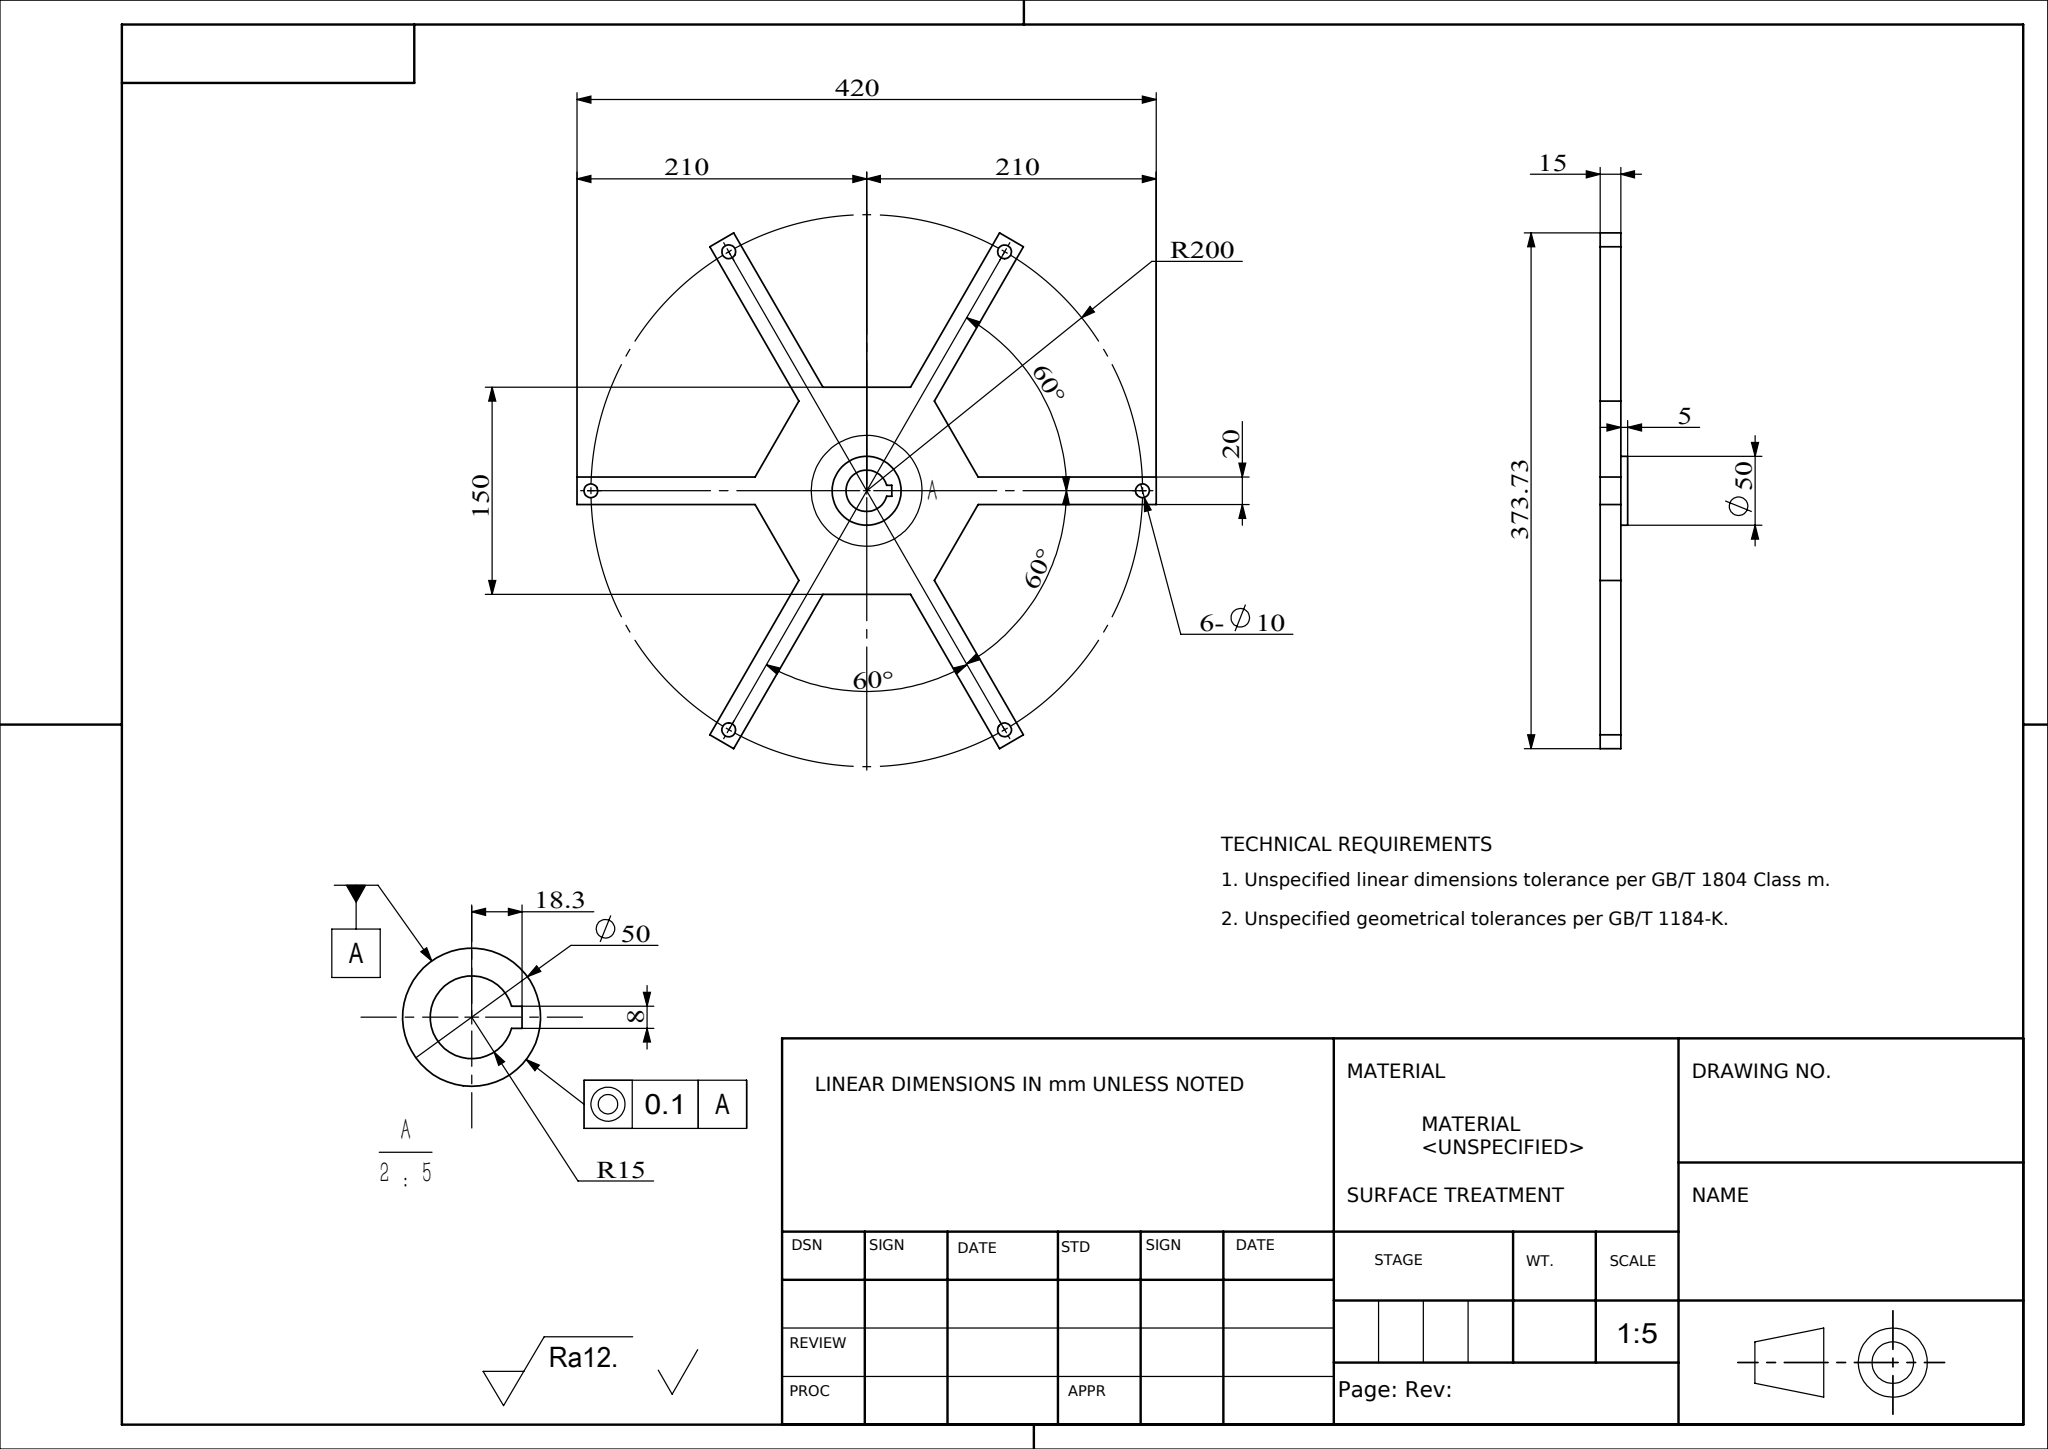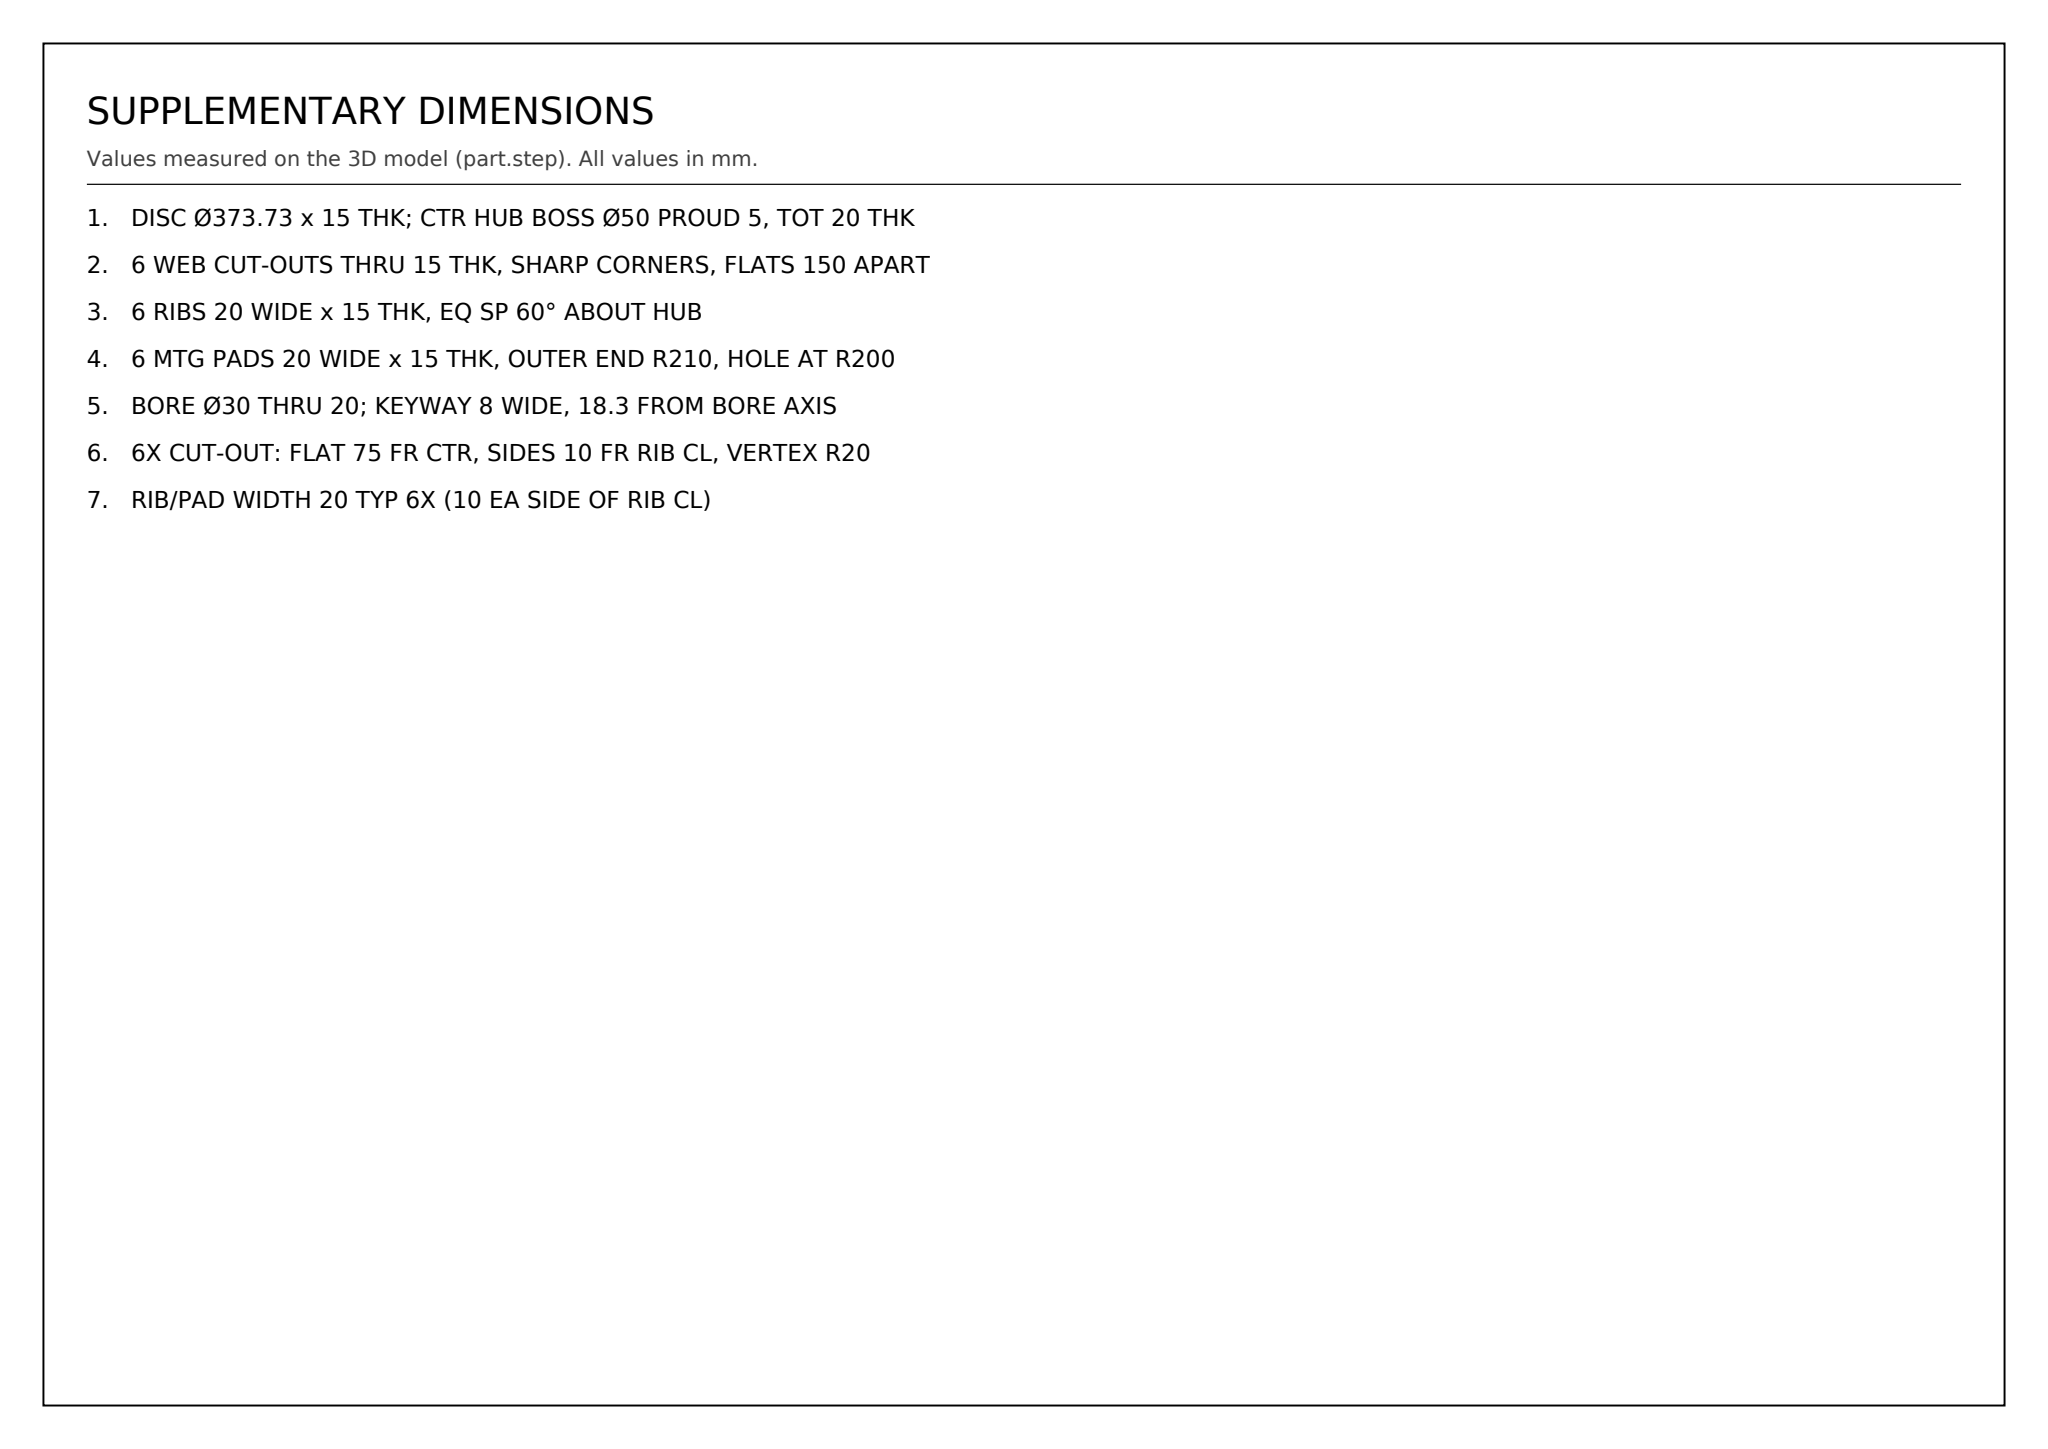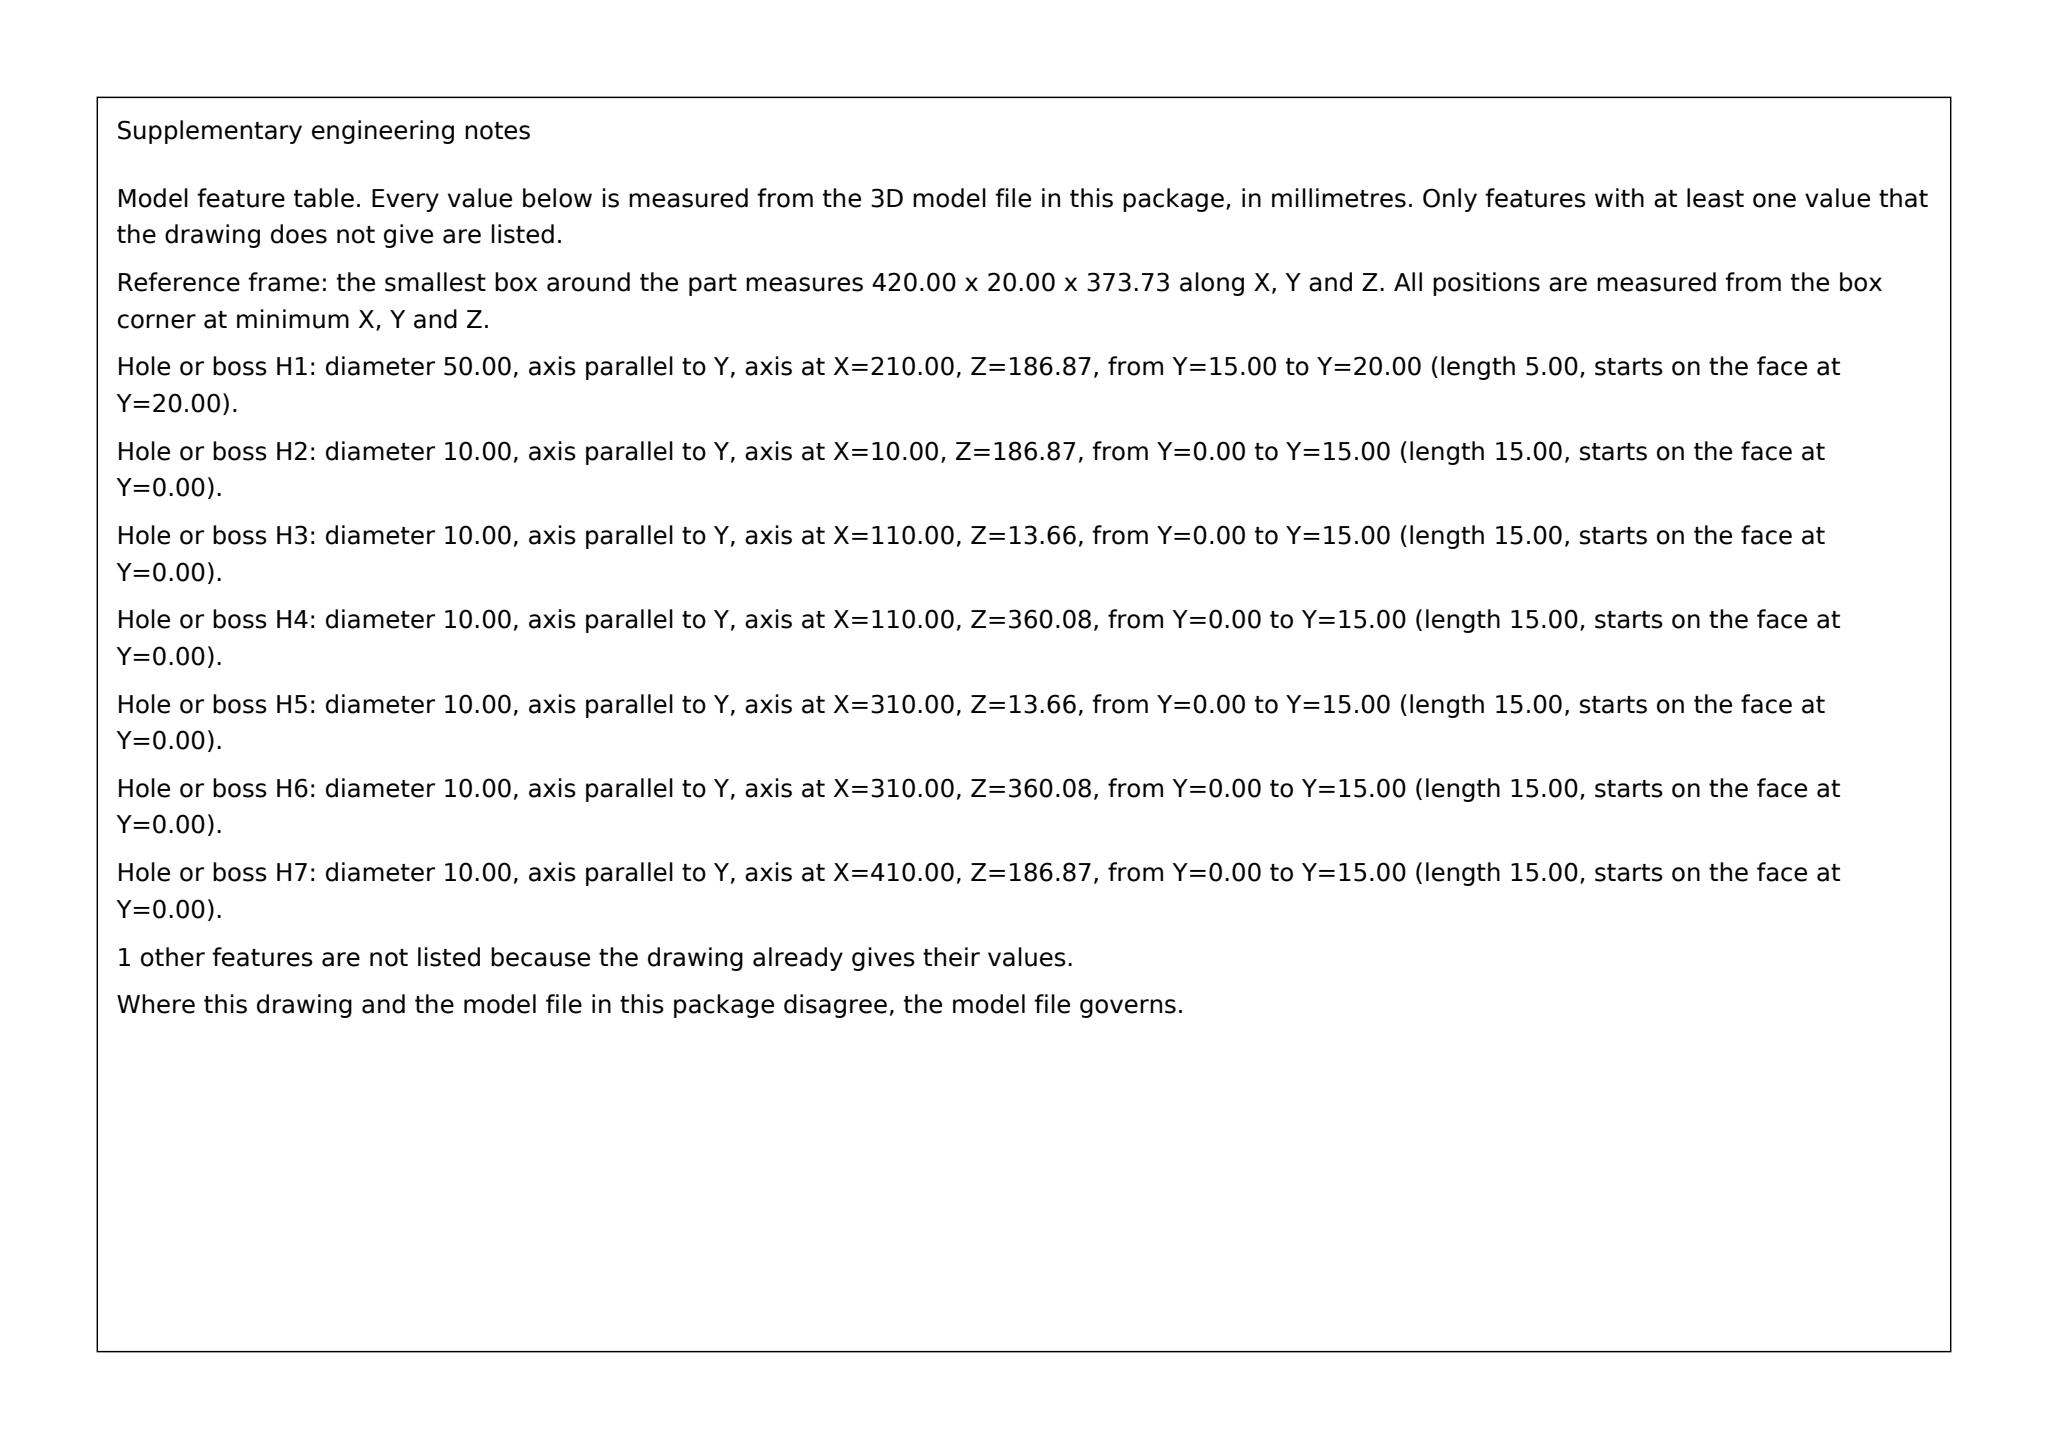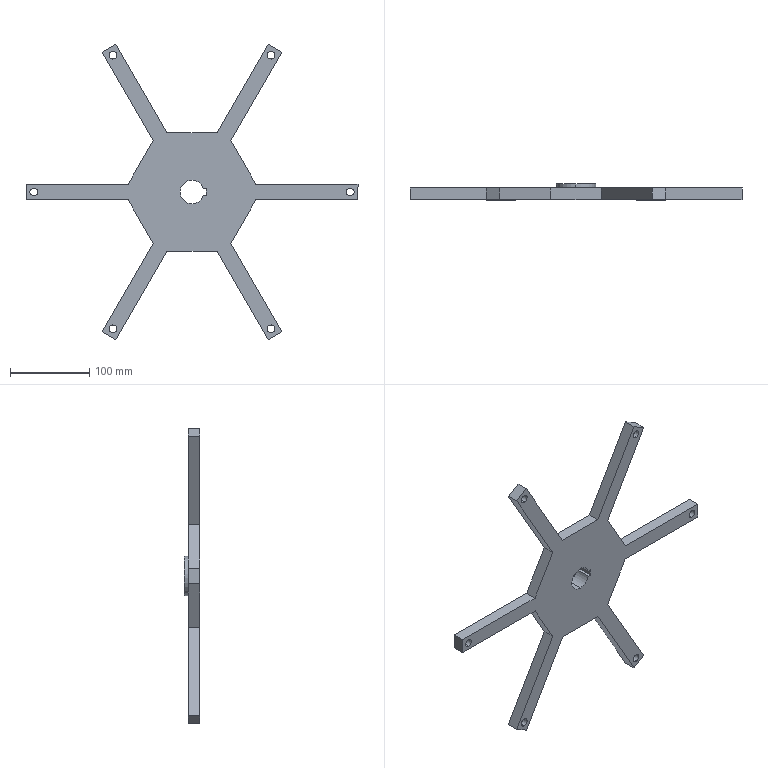Part | SolidWorks | mm | 1 solid | 47 faces | box 420 x 20 x 373.73 mm | volume 507650 mm3 | plane 30 | cylinder 17 | commonest cylinder face diameters 10 x12 30 x3 50 x2
Drawing notes:
DISC Ø373.73 x 15 THK; CTR HUB BOSS Ø50 PROUD 5, TOT 20 THK | from the solid: bbox z=373.731 = disc OD; y planes 0/15/20, bbox y=20; cyl Ø50 axis y len 5 at (210,186.87)
6 WEB CUT-OUTS THRU 15 THK, SHARP CORNERS, FLATS 150 APART | from the solid: fillet_radii [] (no radii); z planes 111.87 & 261.87 = 150 apart, sym about z=186.87; plate 15 thk (y 0-15)
6 RIBS 20 WIDE x 15 THK, EQ SP 60° ABOUT HUB | from the solid: z planes 176.87 & 196.87 straddle rib CL z=186.87 (20 wide); y planes 0/15 = 15 thk; 6-fold Ø10 hole pattern at 60°
6 MTG PADS 20 WIDE x 15 THK, OUTER END R210, HOLE AT R200 | from the solid: pad side planes z=176.87/196.87 (20 wide); x plane 420 = 210 from CL x=210; Ø10 holes at R200 from (210,186.87)
BORE Ø30 THRU 20; KEYWAY 8 WIDE, 18.3 FROM BORE AXIS | from the solid: cyl Ø30 (R15) axis y len 20; keyway faces z=182.87/190.87 (8 wide); end plane x=228.3 = 18.3 from axis x=210
6X CUT-OUT: FLAT 75 FR CTR, SIDES 10 FR RIB CL, VERTEX R20 | from the solid: z planes 111.87 & 261.87 = +/-75 from hub CL z=186.87 (150 apart); z planes 176.87/196.87 = +/-10 from rib CL; ribs 60 deg apart -> inner vertex at R20
RIB/PAD WIDTH 20 TYP 6X (10 EA SIDE OF RIB CL) | from the solid: axis_planes z 176.87 & 196.87 (count 2 each) = 20 wide about hub CL z=186.87; 6 ribs to 6X dia10 holes at R200
build123d program:
from build123d import *

# Parameters (mm, degrees)
BOSS_EXTRUDE1_DEPTH = 15
SKETCH2_R           = 15
CUT_EXTRUDE1_DEPTH  = 20
BOSS_EXTRUDE2_DEPTH = 15
SKETCH4_R           = 5
CUT_EXTRUDE2_DEPTH  = 20
CIRPATTERN1_COUNT   = 6
BOSS_EXTRUDE3_START = 5
SKETCH5_R           = 25
SKETCH5_R_2         = 15
BOSS_EXTRUDE3_DEPTH = 5
SKETCH6_W           = 18.3
SKETCH6_H           = 8
CUT_EXTRUDE3_DEPTH  = 282.813


with BuildPart() as part:
    # Sketch1 → Boss-Extrude1 (new body)
    with BuildSketch(Plane(origin=(0, 0, 0), x_dir=(1, 0, 0), z_dir=(0, 1, 0))):
        Polygon((86.603, 0), (43.301, 75), (-43.301, 75), (-86.603, 0), (-43.301, -75), (43.301, -75), align=None)
    extrude(amount=BOSS_EXTRUDE1_DEPTH)

    # Sketch2 → Cut-Extrude1 (cut)
    with BuildSketch(Plane(origin=(0, 15, 0), x_dir=(1, 0, 0), z_dir=(0, 1, 0))):
        with Locations(Location((0, 0, 0), (0, 0, 270))):
            Circle(SKETCH2_R)
    extrude(amount=-CUT_EXTRUDE1_DEPTH, mode=Mode.SUBTRACT)

    # Sketch3 → Boss-Extrude2 (add)
    with BuildSketch(Plane(origin=(0, 15, 0), x_dir=(1, 0, 0), z_dir=(0, 1, 0))):
        Polygon((24.096, 61.736), (96.34, 186.865), (113.66, 176.865), (41.417, 51.736), align=None)
    boss_extrude2 = extrude(amount=-BOSS_EXTRUDE2_DEPTH)

    # Sketch4 → Cut-Extrude2 (cut)
    with BuildSketch(Plane(origin=(0, 15, 0), x_dir=(1, 0, 0), z_dir=(0, 1, 0))):
        with Locations(Location((100, 173.205, 0), (0, 0, 270))):
            Circle(SKETCH4_R)
    cut_extrude2 = extrude(amount=-CUT_EXTRUDE2_DEPTH, mode=Mode.SUBTRACT)

    # CirPattern1: Boss-Extrude2, Cut-Extrude2 ×6 about axis
    cirpattern1_axis = Axis((0, 0, 0), (0, 1, 0))
    add([boss_extrude2.rotate(cirpattern1_axis, i * 360 / CIRPATTERN1_COUNT) for i in range(1, CIRPATTERN1_COUNT)])
    add([cut_extrude2.rotate(cirpattern1_axis, i * 360 / CIRPATTERN1_COUNT) for i in range(1, CIRPATTERN1_COUNT)], mode=Mode.SUBTRACT)

    # Sketch5 → Boss-Extrude3 (add)
    with BuildSketch(Plane(origin=(0, 15, 0), x_dir=(1, 0, 0), z_dir=(0, 1, 0)).offset(BOSS_EXTRUDE3_START)):
        with Locations(Location((0, 0, 0), (0, 0, 270))):
            Circle(SKETCH5_R)
        with Locations(Location((0, 0, 0), (0, 0, 270))):
            Circle(SKETCH5_R_2, mode=Mode.SUBTRACT)
    extrude(amount=-BOSS_EXTRUDE3_DEPTH)

    # Sketch6 → Cut-Extrude3 (cut, through all)
    with BuildSketch(Plane(origin=(0, 20, 0), x_dir=(1, 0, 0), z_dir=(0, 1, 0))):
        with Locations((9.15, 0)):
            Rectangle(SKETCH6_W, SKETCH6_H)
    extrude(amount=-CUT_EXTRUDE3_DEPTH, mode=Mode.SUBTRACT)


solid = part.part